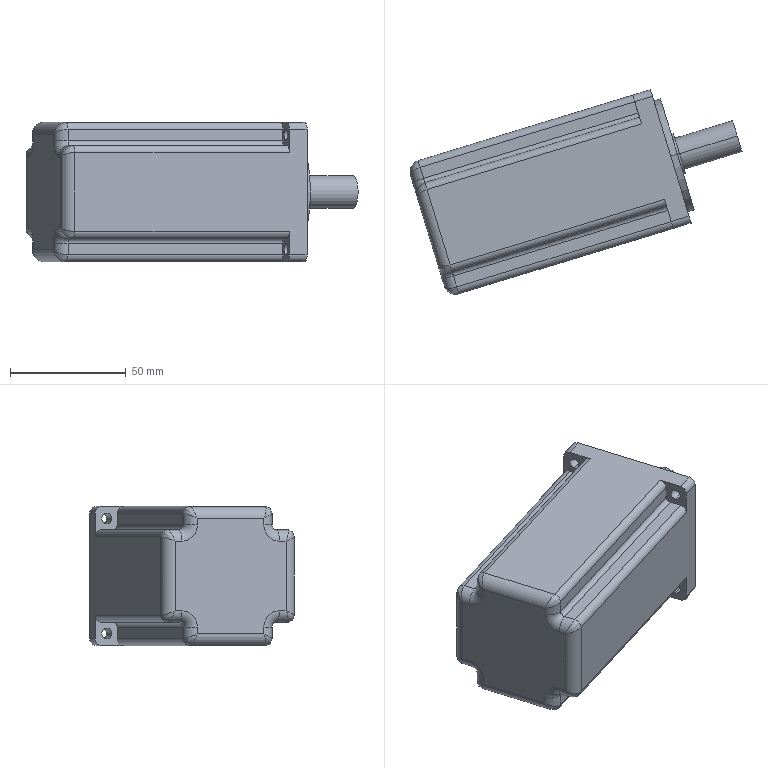Component | SolidWorks | v1ZHXTHG-KR23SB1-1 | 1 solid | 75 faces | box 143.18 x 88.16 x 60 mm | volume 361410 mm3 | cylinder 42 | plane 21 | spline 8 | torus 4 | commonest cylinder face diameters 6 x12 10 x12 4.5 x8 4 x4 14 x2 18 x2 50 x2